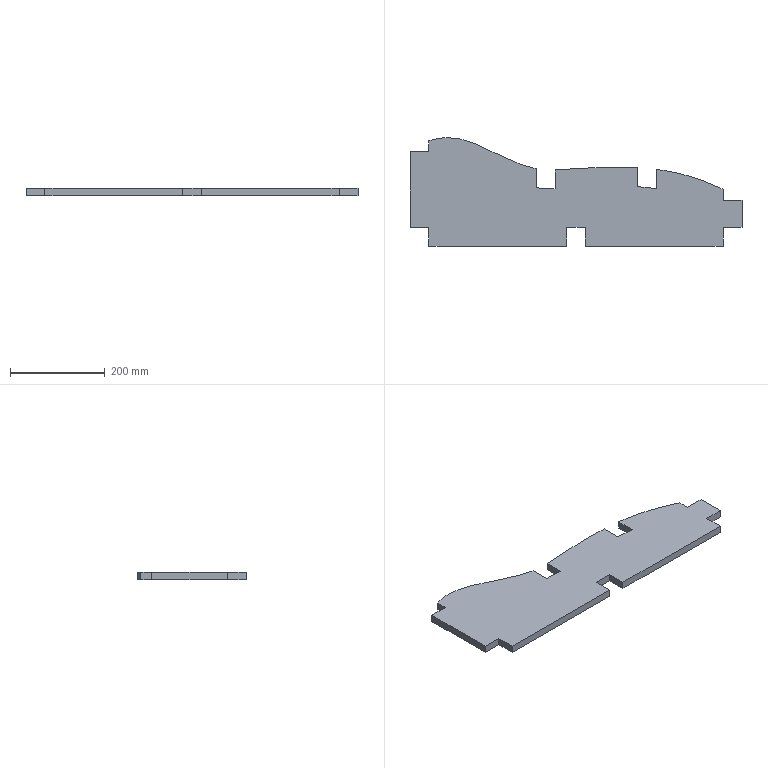Component | SolidWorks | SofaBackrest-1_MiddlePlate-1 | 1 solid | 26 faces | box 700 x 229.46 x 16 mm | volume 1796488 mm3 | plane 23 | spline 3
build123d program:
from build123d import *

# Parameters (mm, degrees)
BOSS_EXTRUDE1_DEPTH = 16


with BuildPart() as part:
    # Sketch1 → Boss-Extrude1 (new body)
    with BuildSketch(Plane.XY):
        with BuildLine():
            Line((-45.794, -11.216), (244.206, -11.216))
            Line((244.206, -11.216), (244.206, 28.784))
            Line((244.206, 28.784), (284.206, 28.784))
            Line((284.206, 28.784), (284.206, -11.216))
            Line((284.206, -11.216), (574.206, -11.216))
            Line((574.206, -11.216), (574.206, 28.784))
            Line((574.206, 28.784), (614.206, 28.784))
            Line((614.206, 28.784), (614.206, 85.912))
            Line((614.206, 85.912), (574.206, 85.912))
            Line((574.206, 85.912), (574.206, 109.398))
            add(Edge.make_bspline(
                [(434.172, 151.119), (482.27, 144.925), (529.206, 132.277), (574.206, 109.398)],
                knots=[0.7358, 0.7358, 0.7358, 0.7358, 0.939, 0.939, 0.939, 0.939], degree=3))
            Line((434.172, 151.119), (434.172, 110.762))
            Line((434.172, 110.762), (394.172, 114.772))
            Line((394.172, 114.772), (394.172, 154.849))
            add(Edge.make_bspline(
                [(220.033, 150.063), (235.562, 150.311), (294.129, 155.332), (352.31, 157.365), (394.172, 154.849)],
                knots=[0.4411, 0.4411, 0.4411, 0.4411, 0.5052, 0.6799, 0.6799, 0.6799, 0.6799], degree=3))
            Line((220.033, 150.063), (220.033, 110.059))
            Line((220.033, 110.059), (180.033, 112.295))
            Line((180.033, 112.295), (180.033, 152.791))
            add(Edge.make_bspline(
                [(-45.794, 211.525), (-17.752, 221.654), (58.249, 214.85), (129.328, 161.794), (180.033, 152.791)],
                knots=[0.05341, 0.05341, 0.05341, 0.05341, 0.1689, 0.3852, 0.3852, 0.3852, 0.3852], degree=3))
            Line((-45.794, 211.525), (-45.794, 188.784))
            Line((-45.794, 188.784), (-85.794, 188.784))
            Line((-85.794, 188.784), (-85.794, 28.784))
            Line((-85.794, 28.784), (-45.794, 28.784))
            Line((-45.794, 28.784), (-45.794, -11.216))
        make_face()
    extrude(amount=BOSS_EXTRUDE1_DEPTH)


solid = part.part

# Placed as in the assembly
solid = solid.moved(Location((97.786, -56.693, 1572), (0, 0, 0)))
STEP:
#1=COLOUR_RGB('',0.7922,0.8196,0.9333);
#2=FILL_AREA_STYLE_COLOUR('',#1);
#3=FILL_AREA_STYLE('',(#2));
#4=SURFACE_STYLE_FILL_AREA(#3);
#5=SURFACE_SIDE_STYLE('',(#4));
#6=SURFACE_STYLE_USAGE(.BOTH.,#5);
#7=PRESENTATION_STYLE_ASSIGNMENT((#6));
#8=CARTESIAN_POINT('',(2.047,5.2,61.89));
#9=VERTEX_POINT('',#8);
#10=CARTESIAN_POINT('',(0.4721,5.2,61.89));
#11=VERTEX_POINT('',#10);
#12=CARTESIAN_POINT('',(0.4721,5.2,61.89));
#13=DIRECTION('',(-1.,0.,0.));
#14=VECTOR('',#13,39.37);
#15=LINE('',#12,#14);
#16=EDGE_CURVE('',#9,#11,#15,.T.);
#17=ORIENTED_EDGE('',*,*,#16,.T.);
#18=CARTESIAN_POINT('',(0.4721,5.2,62.52));
#19=VERTEX_POINT('',#18);
#20=CARTESIAN_POINT('',(0.4721,5.2,62.52));
#21=DIRECTION('',(0.,0.,-1.));
#22=VECTOR('',#21,39.37);
#23=LINE('',#20,#22);
#24=EDGE_CURVE('',#19,#11,#23,.T.);
#25=ORIENTED_EDGE('',*,*,#24,.F.);
#26=CARTESIAN_POINT('',(2.047,5.2,62.52));
#27=VERTEX_POINT('',#26);
#28=CARTESIAN_POINT('',(0.4721,5.2,62.52));
#29=DIRECTION('',(-1.,0.,0.));
#30=VECTOR('',#29,39.37);
#31=LINE('',#28,#30);
#32=EDGE_CURVE('',#27,#19,#31,.T.);
#33=ORIENTED_EDGE('',*,*,#32,.F.);
#34=CARTESIAN_POINT('',(2.047,5.2,62.52));
#35=DIRECTION('',(0.,0.,-1.));
#36=VECTOR('',#35,39.37);
#37=LINE('',#34,#36);
#38=EDGE_CURVE('',#27,#9,#37,.T.);
#39=ORIENTED_EDGE('',*,*,#38,.T.);
#40=EDGE_LOOP('',(#17,#25,#33,#39));
#41=FACE_OUTER_BOUND('',#40,.T.);
#42=CARTESIAN_POINT('',(0.4721,5.2,62.52));
#43=DIRECTION('',(0.,-1.,0.));
#44=DIRECTION('',(0.,0.,-1.));
#45=AXIS2_PLACEMENT_3D('',#42,#43,#44);
#46=PLANE('',#45);
#47=ADVANCED_FACE('',(#41),#46,.F.);
#48=CARTESIAN_POINT('',(0.4721,-1.099,61.89));
#49=VERTEX_POINT('',#48);
#50=CARTESIAN_POINT('',(0.4721,-1.099,61.89));
#51=DIRECTION('',(0.,-1.,0.));
#52=VECTOR('',#51,39.37);
#53=LINE('',#50,#52);
#54=EDGE_CURVE('',#11,#49,#53,.T.);
#55=ORIENTED_EDGE('',*,*,#54,.T.);
#56=CARTESIAN_POINT('',(0.4721,-1.099,62.52));
#57=VERTEX_POINT('',#56);
#58=CARTESIAN_POINT('',(0.4721,-1.099,62.52));
#59=DIRECTION('',(0.,0.,-1.));
#60=VECTOR('',#59,39.37);
#61=LINE('',#58,#60);
#62=EDGE_CURVE('',#57,#49,#61,.T.);
#63=ORIENTED_EDGE('',*,*,#62,.F.);
#64=CARTESIAN_POINT('',(0.4721,-1.099,62.52));
#65=DIRECTION('',(0.,-1.,0.));
#66=VECTOR('',#65,39.37);
#67=LINE('',#64,#66);
#68=EDGE_CURVE('',#19,#57,#67,.T.);
#69=ORIENTED_EDGE('',*,*,#68,.F.);
#70=ORIENTED_EDGE('',*,*,#24,.T.);
#71=EDGE_LOOP('',(#55,#63,#69,#70));
#72=FACE_OUTER_BOUND('',#71,.T.);
#73=CARTESIAN_POINT('',(0.4721,-1.099,62.52));
#74=DIRECTION('',(1.,0.,0.));
#75=DIRECTION('',(0.,0.,-1.));
#76=AXIS2_PLACEMENT_3D('',#73,#74,#75);
#77=PLANE('',#76);
#78=ADVANCED_FACE('',(#72),#77,.F.);
#79=CARTESIAN_POINT('',(2.047,-1.099,61.89));
#80=VERTEX_POINT('',#79);
#81=CARTESIAN_POINT('',(0.4721,-1.099,61.89));
#82=DIRECTION('',(1.,0.,0.));
#83=VECTOR('',#82,39.37);
#84=LINE('',#81,#83);
#85=EDGE_CURVE('',#49,#80,#84,.T.);
#86=ORIENTED_EDGE('',*,*,#85,.T.);
#87=CARTESIAN_POINT('',(2.047,-1.099,62.52));
#88=VERTEX_POINT('',#87);
#89=CARTESIAN_POINT('',(2.047,-1.099,62.52));
#90=DIRECTION('',(0.,0.,-1.));
#91=VECTOR('',#90,39.37);
#92=LINE('',#89,#91);
#93=EDGE_CURVE('',#88,#80,#92,.T.);
#94=ORIENTED_EDGE('',*,*,#93,.F.);
#95=CARTESIAN_POINT('',(0.4721,-1.099,62.52));
#96=DIRECTION('',(1.,0.,0.));
#97=VECTOR('',#96,39.37);
#98=LINE('',#95,#97);
#99=EDGE_CURVE('',#57,#88,#98,.T.);
#100=ORIENTED_EDGE('',*,*,#99,.F.);
#101=ORIENTED_EDGE('',*,*,#62,.T.);
#102=EDGE_LOOP('',(#86,#94,#100,#101));
#103=FACE_OUTER_BOUND('',#102,.T.);
#104=CARTESIAN_POINT('',(0.4721,-1.099,62.52));
#105=DIRECTION('',(0.,1.,0.));
#106=DIRECTION('',(0.,0.,1.));
#107=AXIS2_PLACEMENT_3D('',#104,#105,#106);
#108=PLANE('',#107);
#109=ADVANCED_FACE('',(#103),#108,.F.);
#110=CARTESIAN_POINT('',(2.047,-2.674,61.89));
#111=VERTEX_POINT('',#110);
#112=CARTESIAN_POINT('',(2.047,-1.099,61.89));
#113=DIRECTION('',(0.,-1.,0.));
#114=VECTOR('',#113,39.37);
#115=LINE('',#112,#114);
#116=EDGE_CURVE('',#80,#111,#115,.T.);
#117=ORIENTED_EDGE('',*,*,#116,.T.);
#118=CARTESIAN_POINT('',(2.047,-2.674,62.52));
#119=VERTEX_POINT('',#118);
#120=CARTESIAN_POINT('',(2.047,-2.674,62.52));
#121=DIRECTION('',(0.,0.,-1.));
#122=VECTOR('',#121,39.37);
#123=LINE('',#120,#122);
#124=EDGE_CURVE('',#119,#111,#123,.T.);
#125=ORIENTED_EDGE('',*,*,#124,.F.);
#126=CARTESIAN_POINT('',(2.047,-1.099,62.52));
#127=DIRECTION('',(0.,-1.,0.));
#128=VECTOR('',#127,39.37);
#129=LINE('',#126,#128);
#130=EDGE_CURVE('',#88,#119,#129,.T.);
#131=ORIENTED_EDGE('',*,*,#130,.F.);
#132=ORIENTED_EDGE('',*,*,#93,.T.);
#133=EDGE_LOOP('',(#117,#125,#131,#132));
#134=FACE_OUTER_BOUND('',#133,.T.);
#135=CARTESIAN_POINT('',(2.047,-1.099,62.52));
#136=DIRECTION('',(1.,0.,0.));
#137=DIRECTION('',(0.,0.,-1.));
#138=AXIS2_PLACEMENT_3D('',#135,#136,#137);
#139=PLANE('',#138);
#140=ADVANCED_FACE('',(#134),#139,.F.);
#141=CARTESIAN_POINT('',(13.464,-2.674,61.89));
#142=VERTEX_POINT('',#141);
#143=CARTESIAN_POINT('',(2.047,-2.674,61.89));
#144=DIRECTION('',(1.,0.,0.));
#145=VECTOR('',#144,39.37);
#146=LINE('',#143,#145);
#147=EDGE_CURVE('',#111,#142,#146,.T.);
#148=ORIENTED_EDGE('',*,*,#147,.T.);
#149=CARTESIAN_POINT('',(13.464,-2.674,62.52));
#150=VERTEX_POINT('',#149);
#151=CARTESIAN_POINT('',(13.464,-2.674,62.52));
#152=DIRECTION('',(0.,0.,-1.));
#153=VECTOR('',#152,39.37);
#154=LINE('',#151,#153);
#155=EDGE_CURVE('',#150,#142,#154,.T.);
#156=ORIENTED_EDGE('',*,*,#155,.F.);
#157=CARTESIAN_POINT('',(2.047,-2.674,62.52));
#158=DIRECTION('',(1.,0.,0.));
#159=VECTOR('',#158,39.37);
#160=LINE('',#157,#159);
#161=EDGE_CURVE('',#119,#150,#160,.T.);
#162=ORIENTED_EDGE('',*,*,#161,.F.);
#163=ORIENTED_EDGE('',*,*,#124,.T.);
#164=EDGE_LOOP('',(#148,#156,#162,#163));
#165=FACE_OUTER_BOUND('',#164,.T.);
#166=CARTESIAN_POINT('',(2.047,-2.674,62.52));
#167=DIRECTION('',(0.,1.,0.));
#168=DIRECTION('',(0.,0.,1.));
#169=AXIS2_PLACEMENT_3D('',#166,#167,#168);
#170=PLANE('',#169);
#171=ADVANCED_FACE('',(#165),#170,.F.);
#172=CARTESIAN_POINT('',(13.464,-1.099,61.89));
#173=VERTEX_POINT('',#172);
#174=CARTESIAN_POINT('',(13.464,-2.674,61.89));
#175=DIRECTION('',(0.,1.,0.));
#176=VECTOR('',#175,39.37);
#177=LINE('',#174,#176);
#178=EDGE_CURVE('',#142,#173,#177,.T.);
#179=ORIENTED_EDGE('',*,*,#178,.T.);
#180=CARTESIAN_POINT('',(13.464,-1.099,62.52));
#181=VERTEX_POINT('',#180);
#182=CARTESIAN_POINT('',(13.464,-1.099,62.52));
#183=DIRECTION('',(0.,0.,-1.));
#184=VECTOR('',#183,39.37);
#185=LINE('',#182,#184);
#186=EDGE_CURVE('',#181,#173,#185,.T.);
#187=ORIENTED_EDGE('',*,*,#186,.F.);
#188=CARTESIAN_POINT('',(13.464,-2.674,62.52));
#189=DIRECTION('',(0.,1.,0.));
#190=VECTOR('',#189,39.37);
#191=LINE('',#188,#190);
#192=EDGE_CURVE('',#150,#181,#191,.T.);
#193=ORIENTED_EDGE('',*,*,#192,.F.);
#194=ORIENTED_EDGE('',*,*,#155,.T.);
#195=EDGE_LOOP('',(#179,#187,#193,#194));
#196=FACE_OUTER_BOUND('',#195,.T.);
#197=CARTESIAN_POINT('',(13.464,-2.674,62.52));
#198=DIRECTION('',(-1.,0.,0.));
#199=DIRECTION('',(0.,0.,1.));
#200=AXIS2_PLACEMENT_3D('',#197,#198,#199);
#201=PLANE('',#200);
#202=ADVANCED_FACE('',(#196),#201,.F.);
#203=CARTESIAN_POINT('',(15.039,-1.099,61.89));
#204=VERTEX_POINT('',#203);
#205=CARTESIAN_POINT('',(13.464,-1.099,61.89));
#206=DIRECTION('',(1.,0.,0.));
#207=VECTOR('',#206,39.37);
#208=LINE('',#205,#207);
#209=EDGE_CURVE('',#173,#204,#208,.T.);
#210=ORIENTED_EDGE('',*,*,#209,.T.);
#211=CARTESIAN_POINT('',(15.039,-1.099,62.52));
#212=VERTEX_POINT('',#211);
#213=CARTESIAN_POINT('',(15.039,-1.099,62.52));
#214=DIRECTION('',(0.,0.,-1.));
#215=VECTOR('',#214,39.37);
#216=LINE('',#213,#215);
#217=EDGE_CURVE('',#212,#204,#216,.T.);
#218=ORIENTED_EDGE('',*,*,#217,.F.);
#219=CARTESIAN_POINT('',(13.464,-1.099,62.52));
#220=DIRECTION('',(1.,0.,0.));
#221=VECTOR('',#220,39.37);
#222=LINE('',#219,#221);
#223=EDGE_CURVE('',#181,#212,#222,.T.);
#224=ORIENTED_EDGE('',*,*,#223,.F.);
#225=ORIENTED_EDGE('',*,*,#186,.T.);
#226=EDGE_LOOP('',(#210,#218,#224,#225));
#227=FACE_OUTER_BOUND('',#226,.T.);
#228=CARTESIAN_POINT('',(13.464,-1.099,62.52));
#229=DIRECTION('',(0.,1.,0.));
#230=DIRECTION('',(0.,0.,1.));
#231=AXIS2_PLACEMENT_3D('',#228,#229,#230);
#232=PLANE('',#231);
#233=ADVANCED_FACE('',(#227),#232,.F.);
#234=CARTESIAN_POINT('',(15.039,-2.674,61.89));
#235=VERTEX_POINT('',#234);
#236=CARTESIAN_POINT('',(15.039,-2.674,61.89));
#237=DIRECTION('',(0.,-1.,0.));
#238=VECTOR('',#237,39.37);
#239=LINE('',#236,#238);
#240=EDGE_CURVE('',#204,#235,#239,.T.);
#241=ORIENTED_EDGE('',*,*,#240,.T.);
#242=CARTESIAN_POINT('',(15.039,-2.674,62.52));
#243=VERTEX_POINT('',#242);
#244=CARTESIAN_POINT('',(15.039,-2.674,62.52));
#245=DIRECTION('',(0.,0.,-1.));
#246=VECTOR('',#245,39.37);
#247=LINE('',#244,#246);
#248=EDGE_CURVE('',#243,#235,#247,.T.);
#249=ORIENTED_EDGE('',*,*,#248,.F.);
#250=CARTESIAN_POINT('',(15.039,-2.674,62.52));
#251=DIRECTION('',(0.,-1.,0.));
#252=VECTOR('',#251,39.37);
#253=LINE('',#250,#252);
#254=EDGE_CURVE('',#212,#243,#253,.T.);
#255=ORIENTED_EDGE('',*,*,#254,.F.);
#256=ORIENTED_EDGE('',*,*,#217,.T.);
#257=EDGE_LOOP('',(#241,#249,#255,#256));
#258=FACE_OUTER_BOUND('',#257,.T.);
#259=CARTESIAN_POINT('',(15.039,-2.674,62.52));
#260=DIRECTION('',(1.,0.,0.));
#261=DIRECTION('',(0.,0.,-1.));
#262=AXIS2_PLACEMENT_3D('',#259,#260,#261);
#263=PLANE('',#262);
#264=ADVANCED_FACE('',(#258),#263,.F.);
#265=CARTESIAN_POINT('',(26.456,-2.674,61.89));
#266=VERTEX_POINT('',#265);
#267=CARTESIAN_POINT('',(15.039,-2.674,61.89));
#268=DIRECTION('',(1.,0.,0.));
#269=VECTOR('',#268,39.37);
#270=LINE('',#267,#269);
#271=EDGE_CURVE('',#235,#266,#270,.T.);
#272=ORIENTED_EDGE('',*,*,#271,.T.);
#273=CARTESIAN_POINT('',(26.456,-2.674,62.52));
#274=VERTEX_POINT('',#273);
#275=CARTESIAN_POINT('',(26.456,-2.674,62.52));
#276=DIRECTION('',(0.,0.,-1.));
#277=VECTOR('',#276,39.37);
#278=LINE('',#275,#277);
#279=EDGE_CURVE('',#274,#266,#278,.T.);
#280=ORIENTED_EDGE('',*,*,#279,.F.);
#281=CARTESIAN_POINT('',(15.039,-2.674,62.52));
#282=DIRECTION('',(1.,0.,0.));
#283=VECTOR('',#282,39.37);
#284=LINE('',#281,#283);
#285=EDGE_CURVE('',#243,#274,#284,.T.);
#286=ORIENTED_EDGE('',*,*,#285,.F.);
#287=ORIENTED_EDGE('',*,*,#248,.T.);
#288=EDGE_LOOP('',(#272,#280,#286,#287));
#289=FACE_OUTER_BOUND('',#288,.T.);
#290=CARTESIAN_POINT('',(15.039,-2.674,62.52));
#291=DIRECTION('',(-0.,1.,0.));
#292=DIRECTION('',(-1.,-0.,0.));
#293=AXIS2_PLACEMENT_3D('',#290,#291,#292);
#294=PLANE('',#293);
#295=ADVANCED_FACE('',(#289),#294,.F.);
#296=CARTESIAN_POINT('',(26.456,-1.099,61.89));
#297=VERTEX_POINT('',#296);
#298=CARTESIAN_POINT('',(26.456,-1.099,61.89));
#299=DIRECTION('',(0.,1.,0.));
#300=VECTOR('',#299,39.37);
#301=LINE('',#298,#300);
#302=EDGE_CURVE('',#266,#297,#301,.T.);
#303=ORIENTED_EDGE('',*,*,#302,.T.);
#304=CARTESIAN_POINT('',(26.456,-1.099,62.52));
#305=VERTEX_POINT('',#304);
#306=CARTESIAN_POINT('',(26.456,-1.099,62.52));
#307=DIRECTION('',(0.,0.,-1.));
#308=VECTOR('',#307,39.37);
#309=LINE('',#306,#308);
#310=EDGE_CURVE('',#305,#297,#309,.T.);
#311=ORIENTED_EDGE('',*,*,#310,.F.);
#312=CARTESIAN_POINT('',(26.456,-1.099,62.52));
#313=DIRECTION('',(0.,1.,0.));
#314=VECTOR('',#313,39.37);
#315=LINE('',#312,#314);
#316=EDGE_CURVE('',#274,#305,#315,.T.);
#317=ORIENTED_EDGE('',*,*,#316,.F.);
#318=ORIENTED_EDGE('',*,*,#279,.T.);
#319=EDGE_LOOP('',(#303,#311,#317,#318));
#320=FACE_OUTER_BOUND('',#319,.T.);
#321=CARTESIAN_POINT('',(26.456,-1.099,62.52));
#322=DIRECTION('',(-1.,0.,0.));
#323=DIRECTION('',(0.,0.,1.));
#324=AXIS2_PLACEMENT_3D('',#321,#322,#323);
#325=PLANE('',#324);
#326=ADVANCED_FACE('',(#320),#325,.F.);
#327=CARTESIAN_POINT('',(28.031,-1.099,61.89));
#328=VERTEX_POINT('',#327);
#329=CARTESIAN_POINT('',(28.031,-1.099,61.89));
#330=DIRECTION('',(1.,0.,0.));
#331=VECTOR('',#330,39.37);
#332=LINE('',#329,#331);
#333=EDGE_CURVE('',#297,#328,#332,.T.);
#334=ORIENTED_EDGE('',*,*,#333,.T.);
#335=CARTESIAN_POINT('',(28.031,-1.099,62.52));
#336=VERTEX_POINT('',#335);
#337=CARTESIAN_POINT('',(28.031,-1.099,62.52));
#338=DIRECTION('',(0.,0.,-1.));
#339=VECTOR('',#338,39.37);
#340=LINE('',#337,#339);
#341=EDGE_CURVE('',#336,#328,#340,.T.);
#342=ORIENTED_EDGE('',*,*,#341,.F.);
#343=CARTESIAN_POINT('',(28.031,-1.099,62.52));
#344=DIRECTION('',(1.,0.,0.));
#345=VECTOR('',#344,39.37);
#346=LINE('',#343,#345);
#347=EDGE_CURVE('',#305,#336,#346,.T.);
#348=ORIENTED_EDGE('',*,*,#347,.F.);
#349=ORIENTED_EDGE('',*,*,#310,.T.);
#350=EDGE_LOOP('',(#334,#342,#348,#349));
#351=FACE_OUTER_BOUND('',#350,.T.);
#352=CARTESIAN_POINT('',(28.031,-1.099,62.52));
#353=DIRECTION('',(-0.,1.,0.));
#354=DIRECTION('',(-1.,-0.,0.));
#355=AXIS2_PLACEMENT_3D('',#352,#353,#354);
#356=PLANE('',#355);
#357=ADVANCED_FACE('',(#351),#356,.F.);
#358=CARTESIAN_POINT('',(28.031,1.15,61.89));
#359=VERTEX_POINT('',#358);
#360=CARTESIAN_POINT('',(28.031,1.15,61.89));
#361=DIRECTION('',(0.,1.,0.));
#362=VECTOR('',#361,39.37);
#363=LINE('',#360,#362);
#364=EDGE_CURVE('',#328,#359,#363,.T.);
#365=ORIENTED_EDGE('',*,*,#364,.T.);
#366=CARTESIAN_POINT('',(28.031,1.15,62.52));
#367=VERTEX_POINT('',#366);
#368=CARTESIAN_POINT('',(28.031,1.15,62.52));
#369=DIRECTION('',(0.,0.,-1.));
#370=VECTOR('',#369,39.37);
#371=LINE('',#368,#370);
#372=EDGE_CURVE('',#367,#359,#371,.T.);
#373=ORIENTED_EDGE('',*,*,#372,.F.);
#374=CARTESIAN_POINT('',(28.031,1.15,62.52));
#375=DIRECTION('',(0.,1.,0.));
#376=VECTOR('',#375,39.37);
#377=LINE('',#374,#376);
#378=EDGE_CURVE('',#336,#367,#377,.T.);
#379=ORIENTED_EDGE('',*,*,#378,.F.);
#380=ORIENTED_EDGE('',*,*,#341,.T.);
#381=EDGE_LOOP('',(#365,#373,#379,#380));
#382=FACE_OUTER_BOUND('',#381,.T.);
#383=CARTESIAN_POINT('',(28.031,1.15,62.52));
#384=DIRECTION('',(-1.,0.,0.));
#385=DIRECTION('',(0.,0.,1.));
#386=AXIS2_PLACEMENT_3D('',#383,#384,#385);
#387=PLANE('',#386);
#388=ADVANCED_FACE('',(#382),#387,.F.);
#389=CARTESIAN_POINT('',(26.456,1.15,61.89));
#390=VERTEX_POINT('',#389);
#391=CARTESIAN_POINT('',(28.031,1.15,61.89));
#392=DIRECTION('',(-1.,0.,0.));
#393=VECTOR('',#392,39.37);
#394=LINE('',#391,#393);
#395=EDGE_CURVE('',#359,#390,#394,.T.);
#396=ORIENTED_EDGE('',*,*,#395,.T.);
#397=CARTESIAN_POINT('',(26.456,1.15,62.52));
#398=VERTEX_POINT('',#397);
#399=CARTESIAN_POINT('',(26.456,1.15,62.52));
#400=DIRECTION('',(0.,0.,-1.));
#401=VECTOR('',#400,39.37);
#402=LINE('',#399,#401);
#403=EDGE_CURVE('',#398,#390,#402,.T.);
#404=ORIENTED_EDGE('',*,*,#403,.F.);
#405=CARTESIAN_POINT('',(28.031,1.15,62.52));
#406=DIRECTION('',(-1.,0.,0.));
#407=VECTOR('',#406,39.37);
#408=LINE('',#405,#407);
#409=EDGE_CURVE('',#367,#398,#408,.T.);
#410=ORIENTED_EDGE('',*,*,#409,.F.);
#411=ORIENTED_EDGE('',*,*,#372,.T.);
#412=EDGE_LOOP('',(#396,#404,#410,#411));
#413=FACE_OUTER_BOUND('',#412,.T.);
#414=CARTESIAN_POINT('',(28.031,1.15,62.52));
#415=DIRECTION('',(0.,-1.,0.));
#416=DIRECTION('',(0.,0.,-1.));
#417=AXIS2_PLACEMENT_3D('',#414,#415,#416);
#418=PLANE('',#417);
#419=ADVANCED_FACE('',(#413),#418,.F.);
#420=CARTESIAN_POINT('',(26.456,2.075,61.89));
#421=VERTEX_POINT('',#420);
#422=CARTESIAN_POINT('',(26.456,1.15,61.89));
#423=DIRECTION('',(0.,1.,0.));
#424=VECTOR('',#423,39.37);
#425=LINE('',#422,#424);
#426=EDGE_CURVE('',#390,#421,#425,.T.);
#427=ORIENTED_EDGE('',*,*,#426,.T.);
#428=CARTESIAN_POINT('',(26.456,2.075,62.52));
#429=VERTEX_POINT('',#428);
#430=CARTESIAN_POINT('',(26.456,2.075,62.52));
#431=DIRECTION('',(0.,0.,-1.));
#432=VECTOR('',#431,39.37);
#433=LINE('',#430,#432);
#434=EDGE_CURVE('',#429,#421,#433,.T.);
#435=ORIENTED_EDGE('',*,*,#434,.F.);
#436=CARTESIAN_POINT('',(26.456,1.15,62.52));
#437=DIRECTION('',(0.,1.,0.));
#438=VECTOR('',#437,39.37);
#439=LINE('',#436,#438);
#440=EDGE_CURVE('',#398,#429,#439,.T.);
#441=ORIENTED_EDGE('',*,*,#440,.F.);
#442=ORIENTED_EDGE('',*,*,#403,.T.);
#443=EDGE_LOOP('',(#427,#435,#441,#442));
#444=FACE_OUTER_BOUND('',#443,.T.);
#445=CARTESIAN_POINT('',(26.456,1.15,62.52));
#446=DIRECTION('',(-1.,0.,0.));
#447=DIRECTION('',(0.,0.,1.));
#448=AXIS2_PLACEMENT_3D('',#445,#446,#447);
#449=PLANE('',#448);
#450=ADVANCED_FACE('',(#444),#449,.F.);
#451=CARTESIAN_POINT('',(20.943,3.718,61.89));
#452=VERTEX_POINT('',#451);
#453=CARTESIAN_POINT('',(26.456,2.075,61.89));
#454=CARTESIAN_POINT('',(24.685,2.976,61.89));
#455=CARTESIAN_POINT('',(22.837,3.474,61.89));
#456=CARTESIAN_POINT('',(20.943,3.718,61.89));
#457=B_SPLINE_CURVE_WITH_KNOTS('',3,(#453,#454,#455,#456),.UNSPECIFIED.,.F.,.F.,(4,4),(0.7358,0.939),.UNSPECIFIED.);
#458=EDGE_CURVE('',#421,#452,#457,.T.);
#459=ORIENTED_EDGE('',*,*,#458,.T.);
#460=CARTESIAN_POINT('',(20.943,3.718,62.52));
#461=VERTEX_POINT('',#460);
#462=CARTESIAN_POINT('',(20.943,3.718,62.52));
#463=DIRECTION('',(0.,0.,-1.));
#464=VECTOR('',#463,39.37);
#465=LINE('',#462,#464);
#466=EDGE_CURVE('',#461,#452,#465,.T.);
#467=ORIENTED_EDGE('',*,*,#466,.F.);
#468=CARTESIAN_POINT('',(26.456,2.075,62.52));
#469=CARTESIAN_POINT('',(24.685,2.976,62.52));
#470=CARTESIAN_POINT('',(22.837,3.474,62.52));
#471=CARTESIAN_POINT('',(20.943,3.718,62.52));
#472=B_SPLINE_CURVE_WITH_KNOTS('',3,(#468,#469,#470,#471),.UNSPECIFIED.,.F.,.F.,(4,4),(0.7358,0.939),.UNSPECIFIED.);
#473=EDGE_CURVE('',#429,#461,#472,.T.);
#474=ORIENTED_EDGE('',*,*,#473,.F.);
#475=ORIENTED_EDGE('',*,*,#434,.T.);
#476=EDGE_LOOP('',(#459,#467,#474,#475));
#477=FACE_OUTER_BOUND('',#476,.T.);
#478=CARTESIAN_POINT('',(26.456,2.075,62.52));
#479=CARTESIAN_POINT('',(26.456,2.075,61.89));
#480=CARTESIAN_POINT('',(24.685,2.976,62.52));
#481=CARTESIAN_POINT('',(24.685,2.976,61.89));
#482=CARTESIAN_POINT('',(22.837,3.474,62.52));
#483=CARTESIAN_POINT('',(22.837,3.474,61.89));
#484=CARTESIAN_POINT('',(20.943,3.718,62.52));
#485=CARTESIAN_POINT('',(20.943,3.718,61.89));
#486=B_SPLINE_SURFACE_WITH_KNOTS('',3,1,((#478,#479),(#480,#481),(#482,#483),(#484,#485)),.UNSPECIFIED.,.F.,.F.,.F.,(4,4),(2,2),(0.7358,0.939),(0.,1.),.UNSPECIFIED.);
#487=ADVANCED_FACE('',(#477),#486,.F.);
#488=CARTESIAN_POINT('',(20.943,2.129,61.89));
#489=VERTEX_POINT('',#488);
#490=CARTESIAN_POINT('',(20.943,3.718,61.89));
#491=DIRECTION('',(0.,-1.,0.));
#492=VECTOR('',#491,39.37);
#493=LINE('',#490,#492);
#494=EDGE_CURVE('',#452,#489,#493,.T.);
#495=ORIENTED_EDGE('',*,*,#494,.T.);
#496=CARTESIAN_POINT('',(20.943,2.129,62.52));
#497=VERTEX_POINT('',#496);
#498=CARTESIAN_POINT('',(20.943,2.129,62.52));
#499=DIRECTION('',(0.,0.,-1.));
#500=VECTOR('',#499,39.37);
#501=LINE('',#498,#500);
#502=EDGE_CURVE('',#497,#489,#501,.T.);
#503=ORIENTED_EDGE('',*,*,#502,.F.);
#504=CARTESIAN_POINT('',(20.943,3.718,62.52));
#505=DIRECTION('',(0.,-1.,0.));
#506=VECTOR('',#505,39.37);
#507=LINE('',#504,#506);
#508=EDGE_CURVE('',#461,#497,#507,.T.);
#509=ORIENTED_EDGE('',*,*,#508,.F.);
#510=ORIENTED_EDGE('',*,*,#466,.T.);
#511=EDGE_LOOP('',(#495,#503,#509,#510));
#512=FACE_OUTER_BOUND('',#511,.T.);
#513=CARTESIAN_POINT('',(20.943,3.718,62.52));
#514=DIRECTION('',(1.,0.,0.));
#515=DIRECTION('',(0.,0.,-1.));
#516=AXIS2_PLACEMENT_3D('',#513,#514,#515);
#517=PLANE('',#516);
#518=ADVANCED_FACE('',(#512),#517,.F.);
#519=CARTESIAN_POINT('',(19.368,2.287,61.89));
#520=VERTEX_POINT('',#519);
#521=CARTESIAN_POINT('',(19.368,2.287,61.89));
#522=DIRECTION('',(-0.995,0.09975,0.));
#523=VECTOR('',#522,39.37);
#524=LINE('',#521,#523);
#525=EDGE_CURVE('',#489,#520,#524,.T.);
#526=ORIENTED_EDGE('',*,*,#525,.T.);
#527=CARTESIAN_POINT('',(19.368,2.287,62.52));
#528=VERTEX_POINT('',#527);
#529=CARTESIAN_POINT('',(19.368,2.287,62.52));
#530=DIRECTION('',(0.,0.,-1.));
#531=VECTOR('',#530,39.37);
#532=LINE('',#529,#531);
#533=EDGE_CURVE('',#528,#520,#532,.T.);
#534=ORIENTED_EDGE('',*,*,#533,.F.);
#535=CARTESIAN_POINT('',(19.368,2.287,62.52));
#536=DIRECTION('',(-0.995,0.09975,0.));
#537=VECTOR('',#536,39.37);
#538=LINE('',#535,#537);
#539=EDGE_CURVE('',#497,#528,#538,.T.);
#540=ORIENTED_EDGE('',*,*,#539,.F.);
#541=ORIENTED_EDGE('',*,*,#502,.T.);
#542=EDGE_LOOP('',(#526,#534,#540,#541));
#543=FACE_OUTER_BOUND('',#542,.T.);
#544=CARTESIAN_POINT('',(19.368,2.287,62.52));
#545=DIRECTION('',(-0.09975,-0.995,0.));
#546=DIRECTION('',(0.995,-0.09975,0.));
#547=AXIS2_PLACEMENT_3D('',#544,#545,#546);
#548=PLANE('',#547);
#549=ADVANCED_FACE('',(#543),#548,.F.);
#550=CARTESIAN_POINT('',(19.368,3.864,61.89));
#551=VERTEX_POINT('',#550);
#552=CARTESIAN_POINT('',(19.368,3.864,61.89));
#553=DIRECTION('',(0.,1.,0.));
#554=VECTOR('',#553,39.37);
#555=LINE('',#552,#554);
#556=EDGE_CURVE('',#520,#551,#555,.T.);
#557=ORIENTED_EDGE('',*,*,#556,.T.);
#558=CARTESIAN_POINT('',(19.368,3.864,62.52));
#559=VERTEX_POINT('',#558);
#560=CARTESIAN_POINT('',(19.368,3.864,62.52));
#561=DIRECTION('',(0.,0.,-1.));
#562=VECTOR('',#561,39.37);
#563=LINE('',#560,#562);
#564=EDGE_CURVE('',#559,#551,#563,.T.);
#565=ORIENTED_EDGE('',*,*,#564,.F.);
#566=CARTESIAN_POINT('',(19.368,3.864,62.52));
#567=DIRECTION('',(0.,1.,0.));
#568=VECTOR('',#567,39.37);
#569=LINE('',#566,#568);
#570=EDGE_CURVE('',#528,#559,#569,.T.);
#571=ORIENTED_EDGE('',*,*,#570,.F.);
#572=ORIENTED_EDGE('',*,*,#533,.T.);
#573=EDGE_LOOP('',(#557,#565,#571,#572));
#574=FACE_OUTER_BOUND('',#573,.T.);
#575=CARTESIAN_POINT('',(19.368,3.864,62.52));
#576=DIRECTION('',(-1.,0.,0.));
#577=DIRECTION('',(0.,0.,1.));
#578=AXIS2_PLACEMENT_3D('',#575,#576,#577);
#579=PLANE('',#578);
#580=ADVANCED_FACE('',(#574),#579,.F.);
#581=CARTESIAN_POINT('',(12.513,3.676,61.89));
#582=VERTEX_POINT('',#581);
#583=CARTESIAN_POINT('',(19.368,3.864,61.89));
#584=CARTESIAN_POINT('',(17.72,3.963,61.89));
#585=CARTESIAN_POINT('',(15.43,3.883,61.89));
#586=CARTESIAN_POINT('',(13.124,3.686,61.89));
#587=CARTESIAN_POINT('',(12.513,3.676,61.89));
#588=B_SPLINE_CURVE_WITH_KNOTS('',3,(#583,#584,#585,#586,#587),.UNSPECIFIED.,.F.,.F.,(4,1,4),(0.4411,0.6158,0.6799),.UNSPECIFIED.);
#589=EDGE_CURVE('',#551,#582,#588,.T.);
#590=ORIENTED_EDGE('',*,*,#589,.T.);
#591=CARTESIAN_POINT('',(12.513,3.676,62.52));
#592=VERTEX_POINT('',#591);
#593=CARTESIAN_POINT('',(12.513,3.676,62.52));
#594=DIRECTION('',(0.,0.,-1.));
#595=VECTOR('',#594,39.37);
#596=LINE('',#593,#595);
#597=EDGE_CURVE('',#592,#582,#596,.T.);
#598=ORIENTED_EDGE('',*,*,#597,.F.);
#599=CARTESIAN_POINT('',(19.368,3.864,62.52));
#600=CARTESIAN_POINT('',(17.72,3.963,62.52));
#601=CARTESIAN_POINT('',(15.43,3.883,62.52));
#602=CARTESIAN_POINT('',(13.124,3.686,62.52));
#603=CARTESIAN_POINT('',(12.513,3.676,62.52));
#604=B_SPLINE_CURVE_WITH_KNOTS('',3,(#599,#600,#601,#602,#603),.UNSPECIFIED.,.F.,.F.,(4,1,4),(0.4411,0.6158,0.6799),.UNSPECIFIED.);
#605=EDGE_CURVE('',#559,#592,#604,.T.);
#606=ORIENTED_EDGE('',*,*,#605,.F.);
#607=ORIENTED_EDGE('',*,*,#564,.T.);
#608=EDGE_LOOP('',(#590,#598,#606,#607));
#609=FACE_OUTER_BOUND('',#608,.T.);
#610=CARTESIAN_POINT('',(19.368,3.864,62.52));
#611=CARTESIAN_POINT('',(19.368,3.864,61.89));
#612=CARTESIAN_POINT('',(17.72,3.963,62.52));
#613=CARTESIAN_POINT('',(17.72,3.963,61.89));
#614=CARTESIAN_POINT('',(15.43,3.883,62.52));
#615=CARTESIAN_POINT('',(15.43,3.883,61.89));
#616=CARTESIAN_POINT('',(13.124,3.686,62.52));
#617=CARTESIAN_POINT('',(13.124,3.686,61.89));
#618=CARTESIAN_POINT('',(12.513,3.676,62.52));
#619=CARTESIAN_POINT('',(12.513,3.676,61.89));
#620=B_SPLINE_SURFACE_WITH_KNOTS('',3,1,((#610,#611),(#612,#613),(#614,#615),(#616,#617),(#618,#619)),.UNSPECIFIED.,.F.,.F.,.F.,(4,1,4),(2,2),(0.4411,0.6158,0.6799),(0.,1.),.UNSPECIFIED.);
#621=ADVANCED_FACE('',(#609),#620,.F.);
#622=CARTESIAN_POINT('',(12.513,2.101,61.89));
#623=VERTEX_POINT('',#622);
#624=CARTESIAN_POINT('',(12.513,3.676,61.89));
#625=DIRECTION('',(0.,-1.,0.));
#626=VECTOR('',#625,39.37);
#627=LINE('',#624,#626);
#628=EDGE_CURVE('',#582,#623,#627,.T.);
#629=ORIENTED_EDGE('',*,*,#628,.T.);
#630=CARTESIAN_POINT('',(12.513,2.101,62.52));
#631=VERTEX_POINT('',#630);
#632=CARTESIAN_POINT('',(12.513,2.101,62.52));
#633=DIRECTION('',(0.,0.,-1.));
#634=VECTOR('',#633,39.37);
#635=LINE('',#632,#634);
#636=EDGE_CURVE('',#631,#623,#635,.T.);
#637=ORIENTED_EDGE('',*,*,#636,.F.);
#638=CARTESIAN_POINT('',(12.513,3.676,62.52));
#639=DIRECTION('',(0.,-1.,0.));
#640=VECTOR('',#639,39.37);
#641=LINE('',#638,#640);
#642=EDGE_CURVE('',#592,#631,#641,.T.);
#643=ORIENTED_EDGE('',*,*,#642,.F.);
#644=ORIENTED_EDGE('',*,*,#597,.T.);
#645=EDGE_LOOP('',(#629,#637,#643,#644));
#646=FACE_OUTER_BOUND('',#645,.T.);
#647=CARTESIAN_POINT('',(12.513,3.676,62.52));
#648=DIRECTION('',(1.,0.,0.));
#649=DIRECTION('',(0.,0.,-1.));
#650=AXIS2_PLACEMENT_3D('',#647,#648,#649);
#651=PLANE('',#650);
#652=ADVANCED_FACE('',(#646),#651,.F.);
#653=CARTESIAN_POINT('',(10.938,2.189,61.89));
#654=VERTEX_POINT('',#653);
#655=CARTESIAN_POINT('',(10.938,2.189,61.89));
#656=DIRECTION('',(-0.9984,0.05582,0.));
#657=VECTOR('',#656,39.37);
#658=LINE('',#655,#657);
#659=EDGE_CURVE('',#623,#654,#658,.T.);
#660=ORIENTED_EDGE('',*,*,#659,.T.);
#661=CARTESIAN_POINT('',(10.938,2.189,62.52));
#662=VERTEX_POINT('',#661);
#663=CARTESIAN_POINT('',(10.938,2.189,62.52));
#664=DIRECTION('',(0.,0.,-1.));
#665=VECTOR('',#664,39.37);
#666=LINE('',#663,#665);
#667=EDGE_CURVE('',#662,#654,#666,.T.);
#668=ORIENTED_EDGE('',*,*,#667,.F.);
#669=CARTESIAN_POINT('',(10.938,2.189,62.52));
#670=DIRECTION('',(-0.9984,0.05582,0.));
#671=VECTOR('',#670,39.37);
#672=LINE('',#669,#671);
#673=EDGE_CURVE('',#631,#662,#672,.T.);
#674=ORIENTED_EDGE('',*,*,#673,.F.);
#675=ORIENTED_EDGE('',*,*,#636,.T.);
#676=EDGE_LOOP('',(#660,#668,#674,#675));
#677=FACE_OUTER_BOUND('',#676,.T.);
#678=CARTESIAN_POINT('',(10.938,2.189,62.52));
#679=DIRECTION('',(-0.05582,-0.9984,0.));
#680=DIRECTION('',(0.9984,-0.05582,0.));
#681=AXIS2_PLACEMENT_3D('',#678,#679,#680);
#682=PLANE('',#681);
#683=ADVANCED_FACE('',(#677),#682,.F.);
#684=CARTESIAN_POINT('',(10.938,3.783,61.89));
#685=VERTEX_POINT('',#684);
#686=CARTESIAN_POINT('',(10.938,3.783,61.89));
#687=DIRECTION('',(0.,1.,0.));
#688=VECTOR('',#687,39.37);
#689=LINE('',#686,#688);
#690=EDGE_CURVE('',#654,#685,#689,.T.);
#691=ORIENTED_EDGE('',*,*,#690,.T.);
#692=CARTESIAN_POINT('',(10.938,3.783,62.52));
#693=VERTEX_POINT('',#692);
#694=CARTESIAN_POINT('',(10.938,3.783,62.52));
#695=DIRECTION('',(0.,0.,-1.));
#696=VECTOR('',#695,39.37);
#697=LINE('',#694,#696);
#698=EDGE_CURVE('',#693,#685,#697,.T.);
#699=ORIENTED_EDGE('',*,*,#698,.F.);
#700=CARTESIAN_POINT('',(10.938,3.783,62.52));
#701=DIRECTION('',(0.,1.,0.));
#702=VECTOR('',#701,39.37);
#703=LINE('',#700,#702);
#704=EDGE_CURVE('',#662,#693,#703,.T.);
#705=ORIENTED_EDGE('',*,*,#704,.F.);
#706=ORIENTED_EDGE('',*,*,#667,.T.);
#707=EDGE_LOOP('',(#691,#699,#705,#706));
#708=FACE_OUTER_BOUND('',#707,.T.);
#709=CARTESIAN_POINT('',(10.938,3.783,62.52));
#710=DIRECTION('',(-1.,0.,0.));
#711=DIRECTION('',(0.,0.,1.));
#712=AXIS2_PLACEMENT_3D('',#709,#710,#711);
#713=PLANE('',#712);
#714=ADVANCED_FACE('',(#708),#713,.F.);
#715=CARTESIAN_POINT('',(2.047,6.096,61.89));
#716=VERTEX_POINT('',#715);
#717=CARTESIAN_POINT('',(10.938,3.783,61.89));
#718=CARTESIAN_POINT('',(8.941,4.138,61.89));
#719=CARTESIAN_POINT('',(6.143,6.227,61.89));
#720=CARTESIAN_POINT('',(3.151,6.495,61.89));
#721=CARTESIAN_POINT('',(2.047,6.096,61.89));
#722=B_SPLINE_CURVE_WITH_KNOTS('',3,(#717,#718,#719,#720,#721),.UNSPECIFIED.,.F.,.F.,(4,1,4),(0.05341,0.2697,0.3852),.UNSPECIFIED.);
#723=EDGE_CURVE('',#685,#716,#722,.T.);
#724=ORIENTED_EDGE('',*,*,#723,.T.);
#725=CARTESIAN_POINT('',(2.047,6.096,62.52));
#726=VERTEX_POINT('',#725);
#727=CARTESIAN_POINT('',(2.047,6.096,62.52));
#728=DIRECTION('',(0.,0.,-1.));
#729=VECTOR('',#728,39.37);
#730=LINE('',#727,#729);
#731=EDGE_CURVE('',#726,#716,#730,.T.);
#732=ORIENTED_EDGE('',*,*,#731,.F.);
#733=CARTESIAN_POINT('',(10.938,3.783,62.52));
#734=CARTESIAN_POINT('',(8.941,4.138,62.52));
#735=CARTESIAN_POINT('',(6.143,6.227,62.52));
#736=CARTESIAN_POINT('',(3.151,6.495,62.52));
#737=CARTESIAN_POINT('',(2.047,6.096,62.52));
#738=B_SPLINE_CURVE_WITH_KNOTS('',3,(#733,#734,#735,#736,#737),.UNSPECIFIED.,.F.,.F.,(4,1,4),(0.05341,0.2697,0.3852),.UNSPECIFIED.);
#739=EDGE_CURVE('',#693,#726,#738,.T.);
#740=ORIENTED_EDGE('',*,*,#739,.F.);
#741=ORIENTED_EDGE('',*,*,#698,.T.);
#742=EDGE_LOOP('',(#724,#732,#740,#741));
#743=FACE_OUTER_BOUND('',#742,.T.);
#744=CARTESIAN_POINT('',(10.938,3.783,62.52));
#745=CARTESIAN_POINT('',(10.938,3.783,61.89));
#746=CARTESIAN_POINT('',(8.941,4.138,62.52));
#747=CARTESIAN_POINT('',(8.941,4.138,61.89));
#748=CARTESIAN_POINT('',(6.143,6.227,62.52));
#749=CARTESIAN_POINT('',(6.143,6.227,61.89));
#750=CARTESIAN_POINT('',(3.151,6.495,62.52));
#751=CARTESIAN_POINT('',(3.151,6.495,61.89));
#752=CARTESIAN_POINT('',(2.047,6.096,62.52));
#753=CARTESIAN_POINT('',(2.047,6.096,61.89));
#754=B_SPLINE_SURFACE_WITH_KNOTS('',3,1,((#744,#745),(#746,#747),(#748,#749),(#750,#751),(#752,#753)),.UNSPECIFIED.,.F.,.F.,.F.,(4,1,4),(2,2),(0.05341,0.2697,0.3852),(0.,1.),.UNSPECIFIED.);
#755=ADVANCED_FACE('',(#743),#754,.F.);
#756=CARTESIAN_POINT('',(2.047,5.2,61.89));
#757=DIRECTION('',(-0.,-1.,0.));
#758=VECTOR('',#757,39.37);
#759=LINE('',#756,#758);
#760=EDGE_CURVE('',#716,#9,#759,.T.);
#761=ORIENTED_EDGE('',*,*,#760,.T.);
#762=ORIENTED_EDGE('',*,*,#38,.F.);
#763=CARTESIAN_POINT('',(2.047,5.2,62.52));
#764=DIRECTION('',(-0.,-1.,0.));
#765=VECTOR('',#764,39.37);
#766=LINE('',#763,#765);
#767=EDGE_CURVE('',#726,#27,#766,.T.);
#768=ORIENTED_EDGE('',*,*,#767,.F.);
#769=ORIENTED_EDGE('',*,*,#731,.T.);
#770=EDGE_LOOP('',(#761,#762,#768,#769));
#771=FACE_OUTER_BOUND('',#770,.T.);
#772=CARTESIAN_POINT('',(2.047,5.2,62.52));
#773=DIRECTION('',(1.,-0.,0.));
#774=DIRECTION('',(0.,1.,0.));
#775=AXIS2_PLACEMENT_3D('',#772,#773,#774);
#776=PLANE('',#775);
#777=ADVANCED_FACE('',(#771),#776,.F.);
#778=ORIENTED_EDGE('',*,*,#32,.T.);
#779=ORIENTED_EDGE('',*,*,#68,.T.);
#780=ORIENTED_EDGE('',*,*,#99,.T.);
#781=ORIENTED_EDGE('',*,*,#130,.T.);
#782=ORIENTED_EDGE('',*,*,#161,.T.);
#783=ORIENTED_EDGE('',*,*,#192,.T.);
#784=ORIENTED_EDGE('',*,*,#223,.T.);
#785=ORIENTED_EDGE('',*,*,#254,.T.);
#786=ORIENTED_EDGE('',*,*,#285,.T.);
#787=ORIENTED_EDGE('',*,*,#316,.T.);
#788=ORIENTED_EDGE('',*,*,#347,.T.);
#789=ORIENTED_EDGE('',*,*,#378,.T.);
#790=ORIENTED_EDGE('',*,*,#409,.T.);
#791=ORIENTED_EDGE('',*,*,#440,.T.);
#792=ORIENTED_EDGE('',*,*,#473,.T.);
#793=ORIENTED_EDGE('',*,*,#508,.T.);
#794=ORIENTED_EDGE('',*,*,#539,.T.);
#795=ORIENTED_EDGE('',*,*,#570,.T.);
#796=ORIENTED_EDGE('',*,*,#605,.T.);
#797=ORIENTED_EDGE('',*,*,#642,.T.);
#798=ORIENTED_EDGE('',*,*,#673,.T.);
#799=ORIENTED_EDGE('',*,*,#704,.T.);
#800=ORIENTED_EDGE('',*,*,#739,.T.);
#801=ORIENTED_EDGE('',*,*,#767,.T.);
#802=EDGE_LOOP('',(#778,#779,#780,#781,#782,#783,#784,#785,#786,#787,#788,#789,#790,#791,#792,#793,#794,#795,#796,#797,#798,#799,#800,#801));
#803=FACE_OUTER_BOUND('',#802,.T.);
#804=CARTESIAN_POINT('',(6.533,5.573,62.52));
#805=DIRECTION('',(0.,0.,1.));
#806=DIRECTION('',(1.,0.,0.));
#807=AXIS2_PLACEMENT_3D('',#804,#805,#806);
#808=PLANE('',#807);
#809=ADVANCED_FACE('',(#803),#808,.T.);
#810=ORIENTED_EDGE('',*,*,#16,.F.);
#811=ORIENTED_EDGE('',*,*,#760,.F.);
#812=ORIENTED_EDGE('',*,*,#723,.F.);
#813=ORIENTED_EDGE('',*,*,#690,.F.);
#814=ORIENTED_EDGE('',*,*,#659,.F.);
#815=ORIENTED_EDGE('',*,*,#628,.F.);
#816=ORIENTED_EDGE('',*,*,#589,.F.);
#817=ORIENTED_EDGE('',*,*,#556,.F.);
#818=ORIENTED_EDGE('',*,*,#525,.F.);
#819=ORIENTED_EDGE('',*,*,#494,.F.);
#820=ORIENTED_EDGE('',*,*,#458,.F.);
#821=ORIENTED_EDGE('',*,*,#426,.F.);
#822=ORIENTED_EDGE('',*,*,#395,.F.);
#823=ORIENTED_EDGE('',*,*,#364,.F.);
#824=ORIENTED_EDGE('',*,*,#333,.F.);
#825=ORIENTED_EDGE('',*,*,#302,.F.);
#826=ORIENTED_EDGE('',*,*,#271,.F.);
#827=ORIENTED_EDGE('',*,*,#240,.F.);
#828=ORIENTED_EDGE('',*,*,#209,.F.);
#829=ORIENTED_EDGE('',*,*,#178,.F.);
#830=ORIENTED_EDGE('',*,*,#147,.F.);
#831=ORIENTED_EDGE('',*,*,#116,.F.);
#832=ORIENTED_EDGE('',*,*,#85,.F.);
#833=ORIENTED_EDGE('',*,*,#54,.F.);
#834=EDGE_LOOP('',(#810,#811,#812,#813,#814,#815,#816,#817,#818,#819,#820,#821,#822,#823,#824,#825,#826,#827,#828,#829,#830,#831,#832,#833));
#835=FACE_OUTER_BOUND('',#834,.T.);
#836=CARTESIAN_POINT('',(6.533,5.573,61.89));
#837=DIRECTION('',(0.,0.,1.));
#838=DIRECTION('',(1.,0.,0.));
#839=AXIS2_PLACEMENT_3D('',#836,#837,#838);
#840=PLANE('',#839);
#841=ADVANCED_FACE('',(#835),#840,.F.);
#842=CLOSED_SHELL('',(#47,#78,#109,#140,#171,#202,#233,#264,#295,#326,#357,#388,#419,#450,#487,#518,#549,#580,#621,#652,#683,#714,#755,#777,#809,#841));
#843=MANIFOLD_SOLID_BREP('',#842);
#844=STYLED_ITEM('',(#7),#843);
#845=(LENGTH_UNIT()NAMED_UNIT(*)SI_UNIT($,.METRE.));
#846=LENGTH_MEASURE_WITH_UNIT(LENGTH_MEASURE(0.0254),#845);
#847=DIMENSIONAL_EXPONENTS(1.,0.,0.,0.,0.,0.,0.);
#848=(CONVERSION_BASED_UNIT('',#846)LENGTH_UNIT()NAMED_UNIT(#847));
#849=UNCERTAINTY_MEASURE_WITH_UNIT(LENGTH_MEASURE(0.00001),#848,'','');
#850=(NAMED_UNIT(*)PLANE_ANGLE_UNIT()SI_UNIT($,.RADIAN.));
#851=(NAMED_UNIT(*)SI_UNIT($,.STERADIAN.)SOLID_ANGLE_UNIT());
#852=(GEOMETRIC_REPRESENTATION_CONTEXT(3)GLOBAL_UNCERTAINTY_ASSIGNED_CONTEXT((#849))GLOBAL_UNIT_ASSIGNED_CONTEXT((#848,#850,#851))REPRESENTATION_CONTEXT('',''));
#853=MECHANICAL_DESIGN_GEOMETRIC_PRESENTATION_REPRESENTATION('',(#844),#852);
#854=CARTESIAN_POINT('',(0.,0.,0.));
#855=DIRECTION('',(0.,0.,1.));
#856=DIRECTION('',(1.,0.,0.));
#857=AXIS2_PLACEMENT_3D('',#854,#855,#856);
#858=(LENGTH_UNIT()NAMED_UNIT(*)SI_UNIT($,.METRE.));
#859=LENGTH_MEASURE_WITH_UNIT(LENGTH_MEASURE(0.0254),#858);
#860=DIMENSIONAL_EXPONENTS(1.,0.,0.,0.,0.,0.,0.);
#861=(CONVERSION_BASED_UNIT('',#859)LENGTH_UNIT()NAMED_UNIT(#860));
#862=UNCERTAINTY_MEASURE_WITH_UNIT(LENGTH_MEASURE(0.00001),#861,'','');
#863=(NAMED_UNIT(*)PLANE_ANGLE_UNIT()SI_UNIT($,.RADIAN.));
#864=(NAMED_UNIT(*)SI_UNIT($,.STERADIAN.)SOLID_ANGLE_UNIT());
#865=(GEOMETRIC_REPRESENTATION_CONTEXT(3)GLOBAL_UNCERTAINTY_ASSIGNED_CONTEXT((#862))GLOBAL_UNIT_ASSIGNED_CONTEXT((#861,#863,#864))REPRESENTATION_CONTEXT('',''));
#866=ADVANCED_BREP_SHAPE_REPRESENTATION('',(#843,#857),#865);
#867=PRESENTATION_LAYER_ASSIGNMENT('','',(#844));